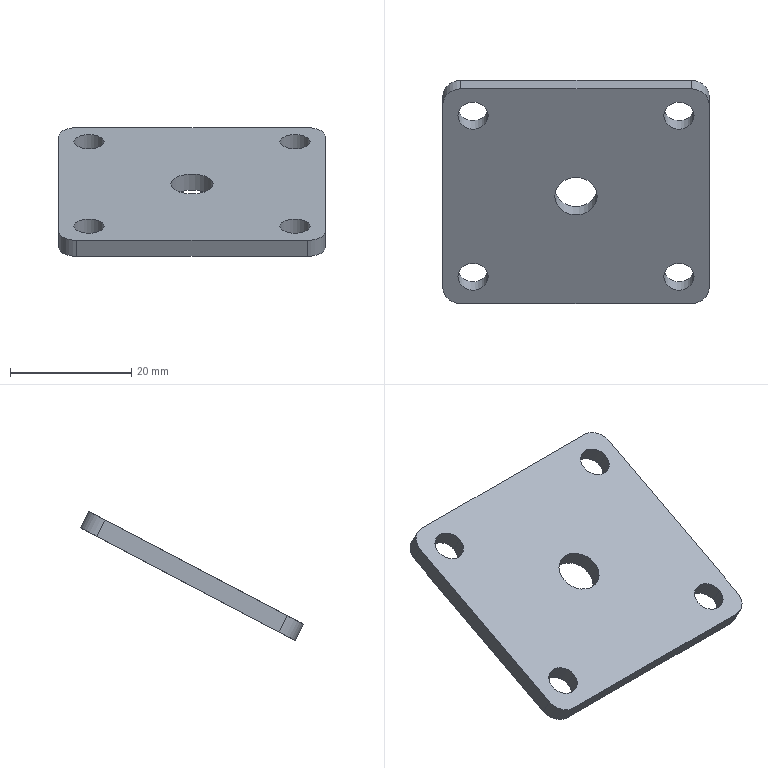Component | SolidWorks | SDACylinderPushPlate-1 | 1 solid | 20 faces | box 44 x 36.81 x 21.25 mm | volume 4906 mm3 | cylinder 14 | plane 6 | commonest cylinder face diameters 5 x8 6 x4 7 x2
STEP:
#1=COLOUR_RGB('',0.7922,0.8196,0.9333);
#2=FILL_AREA_STYLE_COLOUR('',#1);
#3=FILL_AREA_STYLE('',(#2));
#4=SURFACE_STYLE_FILL_AREA(#3);
#5=SURFACE_SIDE_STYLE('',(#4));
#6=SURFACE_STYLE_USAGE(.BOTH.,#5);
#7=PRESENTATION_STYLE_ASSIGNMENT((#6));
#8=CARTESIAN_POINT('',(-9.087,0.1913,6.018));
#9=VERTEX_POINT('',#8);
#10=CARTESIAN_POINT('',(-8.89,0.1913,6.018));
#11=VERTEX_POINT('',#10);
#12=CARTESIAN_POINT('',(-8.989,0.1913,6.018));
#13=DIRECTION('',(0.,-0.4648,0.8854));
#14=DIRECTION('',(1.,0.,0.));
#15=AXIS2_PLACEMENT_3D('',#12,#13,#14);
#16=CIRCLE('',#15,0.09843);
#17=EDGE_CURVE('',#9,#11,#16,.T.);
#18=ORIENTED_EDGE('',*,*,#17,.T.);
#19=CARTESIAN_POINT('',(-8.89,0.2462,5.913));
#20=VERTEX_POINT('',#19);
#21=CARTESIAN_POINT('',(-8.89,0.2462,5.913));
#22=DIRECTION('',(-0.,0.4648,-0.8854));
#23=VECTOR('',#22,39.37);
#24=LINE('',#21,#23);
#25=EDGE_CURVE('',#11,#20,#24,.T.);
#26=ORIENTED_EDGE('',*,*,#25,.T.);
#27=CARTESIAN_POINT('',(-9.087,0.2462,5.913));
#28=VERTEX_POINT('',#27);
#29=CARTESIAN_POINT('',(-8.989,0.2462,5.913));
#30=DIRECTION('',(-0.,0.4648,-0.8854));
#31=DIRECTION('',(-1.,-0.,0.));
#32=AXIS2_PLACEMENT_3D('',#29,#30,#31);
#33=CIRCLE('',#32,0.09843);
#34=EDGE_CURVE('',#20,#28,#33,.T.);
#35=ORIENTED_EDGE('',*,*,#34,.T.);
#36=CARTESIAN_POINT('',(-9.087,0.2462,5.913));
#37=DIRECTION('',(-0.,0.4648,-0.8854));
#38=VECTOR('',#37,39.37);
#39=LINE('',#36,#38);
#40=EDGE_CURVE('',#9,#28,#39,.T.);
#41=ORIENTED_EDGE('',*,*,#40,.F.);
#42=EDGE_LOOP('',(#18,#26,#35,#41));
#43=FACE_OUTER_BOUND('',#42,.T.);
#44=CARTESIAN_POINT('',(-8.989,0.2462,5.913));
#45=DIRECTION('',(-0.,0.4648,-0.8854));
#46=DIRECTION('',(-1.,-0.,0.));
#47=AXIS2_PLACEMENT_3D('',#44,#45,#46);
#48=CYLINDRICAL_SURFACE('',#47,0.09843);
#49=ADVANCED_FACE('',(#43),#48,.F.);
#50=CARTESIAN_POINT('',(-10.426,0.1913,6.018));
#51=VERTEX_POINT('',#50);
#52=CARTESIAN_POINT('',(-10.229,0.1913,6.018));
#53=VERTEX_POINT('',#52);
#54=CARTESIAN_POINT('',(-10.327,0.1913,6.018));
#55=DIRECTION('',(0.,-0.4648,0.8854));
#56=DIRECTION('',(1.,0.,0.));
#57=AXIS2_PLACEMENT_3D('',#54,#55,#56);
#58=CIRCLE('',#57,0.09843);
#59=EDGE_CURVE('',#51,#53,#58,.T.);
#60=ORIENTED_EDGE('',*,*,#59,.T.);
#61=CARTESIAN_POINT('',(-10.229,0.2462,5.913));
#62=VERTEX_POINT('',#61);
#63=CARTESIAN_POINT('',(-10.229,0.2462,5.913));
#64=DIRECTION('',(-0.,0.4648,-0.8854));
#65=VECTOR('',#64,39.37);
#66=LINE('',#63,#65);
#67=EDGE_CURVE('',#53,#62,#66,.T.);
#68=ORIENTED_EDGE('',*,*,#67,.T.);
#69=CARTESIAN_POINT('',(-10.426,0.2462,5.913));
#70=VERTEX_POINT('',#69);
#71=CARTESIAN_POINT('',(-10.327,0.2462,5.913));
#72=DIRECTION('',(-0.,0.4648,-0.8854));
#73=DIRECTION('',(-1.,-0.,0.));
#74=AXIS2_PLACEMENT_3D('',#71,#72,#73);
#75=CIRCLE('',#74,0.09843);
#76=EDGE_CURVE('',#62,#70,#75,.T.);
#77=ORIENTED_EDGE('',*,*,#76,.T.);
#78=CARTESIAN_POINT('',(-10.426,0.2462,5.913));
#79=DIRECTION('',(-0.,0.4648,-0.8854));
#80=VECTOR('',#79,39.37);
#81=LINE('',#78,#80);
#82=EDGE_CURVE('',#51,#70,#81,.T.);
#83=ORIENTED_EDGE('',*,*,#82,.F.);
#84=EDGE_LOOP('',(#60,#68,#77,#83));
#85=FACE_OUTER_BOUND('',#84,.T.);
#86=CARTESIAN_POINT('',(-10.327,0.2462,5.913));
#87=DIRECTION('',(-0.,0.4648,-0.8854));
#88=DIRECTION('',(-1.,-0.,0.));
#89=AXIS2_PLACEMENT_3D('',#86,#87,#88);
#90=CYLINDRICAL_SURFACE('',#89,0.09843);
#91=ADVANCED_FACE('',(#85),#90,.F.);
#92=CARTESIAN_POINT('',(-9.087,-0.8544,5.469));
#93=VERTEX_POINT('',#92);
#94=CARTESIAN_POINT('',(-8.89,-0.8544,5.469));
#95=VERTEX_POINT('',#94);
#96=CARTESIAN_POINT('',(-8.989,-0.8544,5.469));
#97=DIRECTION('',(0.,-0.4648,0.8854));
#98=DIRECTION('',(1.,0.,0.));
#99=AXIS2_PLACEMENT_3D('',#96,#97,#98);
#100=CIRCLE('',#99,0.09843);
#101=EDGE_CURVE('',#93,#95,#100,.T.);
#102=ORIENTED_EDGE('',*,*,#101,.T.);
#103=CARTESIAN_POINT('',(-8.89,-0.7995,5.364));
#104=VERTEX_POINT('',#103);
#105=CARTESIAN_POINT('',(-8.89,-0.7995,5.364));
#106=DIRECTION('',(-0.,0.4648,-0.8854));
#107=VECTOR('',#106,39.37);
#108=LINE('',#105,#107);
#109=EDGE_CURVE('',#95,#104,#108,.T.);
#110=ORIENTED_EDGE('',*,*,#109,.T.);
#111=CARTESIAN_POINT('',(-9.087,-0.7995,5.364));
#112=VERTEX_POINT('',#111);
#113=CARTESIAN_POINT('',(-8.989,-0.7995,5.364));
#114=DIRECTION('',(-0.,0.4648,-0.8854));
#115=DIRECTION('',(-1.,-0.,0.));
#116=AXIS2_PLACEMENT_3D('',#113,#114,#115);
#117=CIRCLE('',#116,0.09843);
#118=EDGE_CURVE('',#104,#112,#117,.T.);
#119=ORIENTED_EDGE('',*,*,#118,.T.);
#120=CARTESIAN_POINT('',(-9.087,-0.7995,5.364));
#121=DIRECTION('',(-0.,0.4648,-0.8854));
#122=VECTOR('',#121,39.37);
#123=LINE('',#120,#122);
#124=EDGE_CURVE('',#93,#112,#123,.T.);
#125=ORIENTED_EDGE('',*,*,#124,.F.);
#126=EDGE_LOOP('',(#102,#110,#119,#125));
#127=FACE_OUTER_BOUND('',#126,.T.);
#128=CARTESIAN_POINT('',(-8.989,-0.7995,5.364));
#129=DIRECTION('',(-0.,0.4648,-0.8854));
#130=DIRECTION('',(-1.,-0.,0.));
#131=AXIS2_PLACEMENT_3D('',#128,#129,#130);
#132=CYLINDRICAL_SURFACE('',#131,0.09843);
#133=ADVANCED_FACE('',(#127),#132,.F.);
#134=CARTESIAN_POINT('',(-10.426,-0.8544,5.469));
#135=VERTEX_POINT('',#134);
#136=CARTESIAN_POINT('',(-10.229,-0.8544,5.469));
#137=VERTEX_POINT('',#136);
#138=CARTESIAN_POINT('',(-10.327,-0.8544,5.469));
#139=DIRECTION('',(0.,-0.4648,0.8854));
#140=DIRECTION('',(1.,0.,0.));
#141=AXIS2_PLACEMENT_3D('',#138,#139,#140);
#142=CIRCLE('',#141,0.09843);
#143=EDGE_CURVE('',#135,#137,#142,.T.);
#144=ORIENTED_EDGE('',*,*,#143,.T.);
#145=CARTESIAN_POINT('',(-10.229,-0.7995,5.364));
#146=VERTEX_POINT('',#145);
#147=CARTESIAN_POINT('',(-10.229,-0.7995,5.364));
#148=DIRECTION('',(-0.,0.4648,-0.8854));
#149=VECTOR('',#148,39.37);
#150=LINE('',#147,#149);
#151=EDGE_CURVE('',#137,#146,#150,.T.);
#152=ORIENTED_EDGE('',*,*,#151,.T.);
#153=CARTESIAN_POINT('',(-10.426,-0.7995,5.364));
#154=VERTEX_POINT('',#153);
#155=CARTESIAN_POINT('',(-10.327,-0.7995,5.364));
#156=DIRECTION('',(-0.,0.4648,-0.8854));
#157=DIRECTION('',(-1.,-0.,0.));
#158=AXIS2_PLACEMENT_3D('',#155,#156,#157);
#159=CIRCLE('',#158,0.09843);
#160=EDGE_CURVE('',#146,#154,#159,.T.);
#161=ORIENTED_EDGE('',*,*,#160,.T.);
#162=CARTESIAN_POINT('',(-10.426,-0.7995,5.364));
#163=DIRECTION('',(-0.,0.4648,-0.8854));
#164=VECTOR('',#163,39.37);
#165=LINE('',#162,#164);
#166=EDGE_CURVE('',#135,#154,#165,.T.);
#167=ORIENTED_EDGE('',*,*,#166,.F.);
#168=EDGE_LOOP('',(#144,#152,#161,#167));
#169=FACE_OUTER_BOUND('',#168,.T.);
#170=CARTESIAN_POINT('',(-10.327,-0.7995,5.364));
#171=DIRECTION('',(-0.,0.4648,-0.8854));
#172=DIRECTION('',(-1.,-0.,0.));
#173=AXIS2_PLACEMENT_3D('',#170,#171,#172);
#174=CYLINDRICAL_SURFACE('',#173,0.09843);
#175=ADVANCED_FACE('',(#169),#174,.F.);
#176=CARTESIAN_POINT('',(-9.796,-0.3316,5.743));
#177=VERTEX_POINT('',#176);
#178=CARTESIAN_POINT('',(-9.52,-0.3316,5.743));
#179=VERTEX_POINT('',#178);
#180=CARTESIAN_POINT('',(-9.658,-0.3316,5.743));
#181=DIRECTION('',(0.,-0.4648,0.8854));
#182=DIRECTION('',(1.,0.,0.));
#183=AXIS2_PLACEMENT_3D('',#180,#181,#182);
#184=CIRCLE('',#183,0.1378);
#185=EDGE_CURVE('',#177,#179,#184,.T.);
#186=ORIENTED_EDGE('',*,*,#185,.T.);
#187=CARTESIAN_POINT('',(-9.52,-0.2767,5.638));
#188=VERTEX_POINT('',#187);
#189=CARTESIAN_POINT('',(-9.52,-0.2767,5.638));
#190=DIRECTION('',(-0.,0.4648,-0.8854));
#191=VECTOR('',#190,39.37);
#192=LINE('',#189,#191);
#193=EDGE_CURVE('',#179,#188,#192,.T.);
#194=ORIENTED_EDGE('',*,*,#193,.T.);
#195=CARTESIAN_POINT('',(-9.796,-0.2767,5.638));
#196=VERTEX_POINT('',#195);
#197=CARTESIAN_POINT('',(-9.658,-0.2767,5.638));
#198=DIRECTION('',(-0.,0.4648,-0.8854));
#199=DIRECTION('',(-1.,-0.,0.));
#200=AXIS2_PLACEMENT_3D('',#197,#198,#199);
#201=CIRCLE('',#200,0.1378);
#202=EDGE_CURVE('',#188,#196,#201,.T.);
#203=ORIENTED_EDGE('',*,*,#202,.T.);
#204=CARTESIAN_POINT('',(-9.796,-0.2767,5.638));
#205=DIRECTION('',(-0.,0.4648,-0.8854));
#206=VECTOR('',#205,39.37);
#207=LINE('',#204,#206);
#208=EDGE_CURVE('',#177,#196,#207,.T.);
#209=ORIENTED_EDGE('',*,*,#208,.F.);
#210=EDGE_LOOP('',(#186,#194,#203,#209));
#211=FACE_OUTER_BOUND('',#210,.T.);
#212=CARTESIAN_POINT('',(-9.658,-0.2767,5.638));
#213=DIRECTION('',(-0.,0.4648,-0.8854));
#214=DIRECTION('',(-1.,-0.,0.));
#215=AXIS2_PLACEMENT_3D('',#212,#213,#214);
#216=CYLINDRICAL_SURFACE('',#215,0.1378);
#217=ADVANCED_FACE('',(#211),#216,.F.);
#218=CARTESIAN_POINT('',(-10.524,-0.9242,5.432));
#219=VERTEX_POINT('',#218);
#220=CARTESIAN_POINT('',(-10.524,0.261,6.054));
#221=VERTEX_POINT('',#220);
#222=CARTESIAN_POINT('',(-10.524,-1.029,5.377));
#223=DIRECTION('',(-0.,0.8854,0.4648));
#224=VECTOR('',#223,39.37);
#225=LINE('',#222,#224);
#226=EDGE_CURVE('',#219,#221,#225,.T.);
#227=ORIENTED_EDGE('',*,*,#226,.T.);
#228=CARTESIAN_POINT('',(-10.524,0.3159,5.95));
#229=VERTEX_POINT('',#228);
#230=CARTESIAN_POINT('',(-10.524,0.261,6.054));
#231=DIRECTION('',(-0.,0.4648,-0.8854));
#232=VECTOR('',#231,39.37);
#233=LINE('',#230,#232);
#234=EDGE_CURVE('',#221,#229,#233,.T.);
#235=ORIENTED_EDGE('',*,*,#234,.T.);
#236=CARTESIAN_POINT('',(-10.524,-0.8693,5.327));
#237=VERTEX_POINT('',#236);
#238=CARTESIAN_POINT('',(-10.524,-0.9738,5.272));
#239=DIRECTION('',(-0.,0.8854,0.4648));
#240=VECTOR('',#239,39.37);
#241=LINE('',#238,#240);
#242=EDGE_CURVE('',#237,#229,#241,.T.);
#243=ORIENTED_EDGE('',*,*,#242,.F.);
#244=CARTESIAN_POINT('',(-10.524,-0.9242,5.432));
#245=DIRECTION('',(0.,-0.4648,0.8854));
#246=VECTOR('',#245,39.37);
#247=LINE('',#244,#246);
#248=EDGE_CURVE('',#237,#219,#247,.T.);
#249=ORIENTED_EDGE('',*,*,#248,.T.);
#250=EDGE_LOOP('',(#227,#235,#243,#249));
#251=FACE_OUTER_BOUND('',#250,.T.);
#252=CARTESIAN_POINT('',(-10.524,-1.029,5.377));
#253=DIRECTION('',(-1.,-0.,0.));
#254=DIRECTION('',(0.,-0.4648,0.8854));
#255=AXIS2_PLACEMENT_3D('',#252,#253,#254);
#256=PLANE('',#255);
#257=ADVANCED_FACE('',(#251),#256,.T.);
#258=CARTESIAN_POINT('',(-8.91,-1.029,5.377));
#259=VERTEX_POINT('',#258);
#260=CARTESIAN_POINT('',(-10.406,-1.029,5.377));
#261=VERTEX_POINT('',#260);
#262=CARTESIAN_POINT('',(-8.792,-1.029,5.377));
#263=DIRECTION('',(-1.,-0.,0.));
#264=VECTOR('',#263,39.37);
#265=LINE('',#262,#264);
#266=EDGE_CURVE('',#259,#261,#265,.T.);
#267=ORIENTED_EDGE('',*,*,#266,.T.);
#268=CARTESIAN_POINT('',(-10.406,-0.9738,5.272));
#269=VERTEX_POINT('',#268);
#270=CARTESIAN_POINT('',(-10.406,-1.029,5.377));
#271=DIRECTION('',(-0.,0.4648,-0.8854));
#272=VECTOR('',#271,39.37);
#273=LINE('',#270,#272);
#274=EDGE_CURVE('',#261,#269,#273,.T.);
#275=ORIENTED_EDGE('',*,*,#274,.T.);
#276=CARTESIAN_POINT('',(-8.91,-0.9738,5.272));
#277=VERTEX_POINT('',#276);
#278=CARTESIAN_POINT('',(-8.792,-0.9738,5.272));
#279=DIRECTION('',(-1.,-0.,0.));
#280=VECTOR('',#279,39.37);
#281=LINE('',#278,#280);
#282=EDGE_CURVE('',#277,#269,#281,.T.);
#283=ORIENTED_EDGE('',*,*,#282,.F.);
#284=CARTESIAN_POINT('',(-8.91,-1.029,5.377));
#285=DIRECTION('',(0.,-0.4648,0.8854));
#286=VECTOR('',#285,39.37);
#287=LINE('',#284,#286);
#288=EDGE_CURVE('',#277,#259,#287,.T.);
#289=ORIENTED_EDGE('',*,*,#288,.T.);
#290=EDGE_LOOP('',(#267,#275,#283,#289));
#291=FACE_OUTER_BOUND('',#290,.T.);
#292=CARTESIAN_POINT('',(-8.792,-1.029,5.377));
#293=DIRECTION('',(0.,-0.8854,-0.4648));
#294=DIRECTION('',(0.,-0.4648,0.8854));
#295=AXIS2_PLACEMENT_3D('',#292,#293,#294);
#296=PLANE('',#295);
#297=ADVANCED_FACE('',(#291),#296,.T.);
#298=CARTESIAN_POINT('',(-8.792,0.261,6.054));
#299=VERTEX_POINT('',#298);
#300=CARTESIAN_POINT('',(-8.792,-0.9242,5.432));
#301=VERTEX_POINT('',#300);
#302=CARTESIAN_POINT('',(-8.792,-1.029,5.377));
#303=DIRECTION('',(0.,-0.8854,-0.4648));
#304=VECTOR('',#303,39.37);
#305=LINE('',#302,#304);
#306=EDGE_CURVE('',#299,#301,#305,.T.);
#307=ORIENTED_EDGE('',*,*,#306,.T.);
#308=CARTESIAN_POINT('',(-8.792,-0.8693,5.327));
#309=VERTEX_POINT('',#308);
#310=CARTESIAN_POINT('',(-8.792,-0.9242,5.432));
#311=DIRECTION('',(-0.,0.4648,-0.8854));
#312=VECTOR('',#311,39.37);
#313=LINE('',#310,#312);
#314=EDGE_CURVE('',#301,#309,#313,.T.);
#315=ORIENTED_EDGE('',*,*,#314,.T.);
#316=CARTESIAN_POINT('',(-8.792,0.3159,5.95));
#317=VERTEX_POINT('',#316);
#318=CARTESIAN_POINT('',(-8.792,-0.9738,5.272));
#319=DIRECTION('',(0.,-0.8854,-0.4648));
#320=VECTOR('',#319,39.37);
#321=LINE('',#318,#320);
#322=EDGE_CURVE('',#317,#309,#321,.T.);
#323=ORIENTED_EDGE('',*,*,#322,.F.);
#324=CARTESIAN_POINT('',(-8.792,0.261,6.054));
#325=DIRECTION('',(0.,-0.4648,0.8854));
#326=VECTOR('',#325,39.37);
#327=LINE('',#324,#326);
#328=EDGE_CURVE('',#317,#299,#327,.T.);
#329=ORIENTED_EDGE('',*,*,#328,.T.);
#330=EDGE_LOOP('',(#307,#315,#323,#329));
#331=FACE_OUTER_BOUND('',#330,.T.);
#332=CARTESIAN_POINT('',(-8.792,-1.029,5.377));
#333=DIRECTION('',(1.,0.,-0.));
#334=DIRECTION('',(-0.,0.4648,-0.8854));
#335=AXIS2_PLACEMENT_3D('',#332,#333,#334);
#336=PLANE('',#335);
#337=ADVANCED_FACE('',(#331),#336,.T.);
#338=CARTESIAN_POINT('',(-10.406,0.4205,6.004));
#339=VERTEX_POINT('',#338);
#340=CARTESIAN_POINT('',(-8.91,0.4205,6.004));
#341=VERTEX_POINT('',#340);
#342=CARTESIAN_POINT('',(-8.792,0.4205,6.004));
#343=DIRECTION('',(1.,0.,-0.));
#344=VECTOR('',#343,39.37);
#345=LINE('',#342,#344);
#346=EDGE_CURVE('',#339,#341,#345,.T.);
#347=ORIENTED_EDGE('',*,*,#346,.F.);
#348=CARTESIAN_POINT('',(-10.406,0.3656,6.109));
#349=VERTEX_POINT('',#348);
#350=CARTESIAN_POINT('',(-10.406,0.3656,6.109));
#351=DIRECTION('',(0.,-0.4648,0.8854));
#352=VECTOR('',#351,39.37);
#353=LINE('',#350,#352);
#354=EDGE_CURVE('',#339,#349,#353,.T.);
#355=ORIENTED_EDGE('',*,*,#354,.T.);
#356=CARTESIAN_POINT('',(-8.91,0.3656,6.109));
#357=VERTEX_POINT('',#356);
#358=CARTESIAN_POINT('',(-8.792,0.3656,6.109));
#359=DIRECTION('',(1.,0.,-0.));
#360=VECTOR('',#359,39.37);
#361=LINE('',#358,#360);
#362=EDGE_CURVE('',#349,#357,#361,.T.);
#363=ORIENTED_EDGE('',*,*,#362,.T.);
#364=CARTESIAN_POINT('',(-8.91,0.3656,6.109));
#365=DIRECTION('',(-0.,0.4648,-0.8854));
#366=VECTOR('',#365,39.37);
#367=LINE('',#364,#366);
#368=EDGE_CURVE('',#357,#341,#367,.T.);
#369=ORIENTED_EDGE('',*,*,#368,.T.);
#370=EDGE_LOOP('',(#347,#355,#363,#369));
#371=FACE_OUTER_BOUND('',#370,.T.);
#372=CARTESIAN_POINT('',(-8.792,0.3656,6.109));
#373=DIRECTION('',(-0.,0.8854,0.4648));
#374=DIRECTION('',(-0.,0.4648,-0.8854));
#375=AXIS2_PLACEMENT_3D('',#372,#373,#374);
#376=PLANE('',#375);
#377=ADVANCED_FACE('',(#371),#376,.T.);
#378=ORIENTED_EDGE('',*,*,#17,.F.);
#379=CARTESIAN_POINT('',(-8.989,0.1913,6.018));
#380=DIRECTION('',(0.,-0.4648,0.8854));
#381=DIRECTION('',(1.,0.,0.));
#382=AXIS2_PLACEMENT_3D('',#379,#380,#381);
#383=CIRCLE('',#382,0.09843);
#384=EDGE_CURVE('',#11,#9,#383,.T.);
#385=ORIENTED_EDGE('',*,*,#384,.F.);
#386=EDGE_LOOP('',(#378,#385));
#387=FACE_BOUND('',#386,.T.);
#388=ORIENTED_EDGE('',*,*,#59,.F.);
#389=CARTESIAN_POINT('',(-10.327,0.1913,6.018));
#390=DIRECTION('',(0.,-0.4648,0.8854));
#391=DIRECTION('',(1.,0.,0.));
#392=AXIS2_PLACEMENT_3D('',#389,#390,#391);
#393=CIRCLE('',#392,0.09843);
#394=EDGE_CURVE('',#53,#51,#393,.T.);
#395=ORIENTED_EDGE('',*,*,#394,.F.);
#396=EDGE_LOOP('',(#388,#395));
#397=FACE_BOUND('',#396,.T.);
#398=ORIENTED_EDGE('',*,*,#101,.F.);
#399=CARTESIAN_POINT('',(-8.989,-0.8544,5.469));
#400=DIRECTION('',(0.,-0.4648,0.8854));
#401=DIRECTION('',(1.,0.,0.));
#402=AXIS2_PLACEMENT_3D('',#399,#400,#401);
#403=CIRCLE('',#402,0.09843);
#404=EDGE_CURVE('',#95,#93,#403,.T.);
#405=ORIENTED_EDGE('',*,*,#404,.F.);
#406=EDGE_LOOP('',(#398,#405));
#407=FACE_BOUND('',#406,.T.);
#408=ORIENTED_EDGE('',*,*,#143,.F.);
#409=CARTESIAN_POINT('',(-10.327,-0.8544,5.469));
#410=DIRECTION('',(0.,-0.4648,0.8854));
#411=DIRECTION('',(1.,0.,0.));
#412=AXIS2_PLACEMENT_3D('',#409,#410,#411);
#413=CIRCLE('',#412,0.09843);
#414=EDGE_CURVE('',#137,#135,#413,.T.);
#415=ORIENTED_EDGE('',*,*,#414,.F.);
#416=EDGE_LOOP('',(#408,#415));
#417=FACE_BOUND('',#416,.T.);
#418=ORIENTED_EDGE('',*,*,#185,.F.);
#419=CARTESIAN_POINT('',(-9.658,-0.3316,5.743));
#420=DIRECTION('',(0.,-0.4648,0.8854));
#421=DIRECTION('',(1.,0.,0.));
#422=AXIS2_PLACEMENT_3D('',#419,#420,#421);
#423=CIRCLE('',#422,0.1378);
#424=EDGE_CURVE('',#179,#177,#423,.T.);
#425=ORIENTED_EDGE('',*,*,#424,.F.);
#426=EDGE_LOOP('',(#418,#425));
#427=FACE_BOUND('',#426,.T.);
#428=ORIENTED_EDGE('',*,*,#362,.F.);
#429=CARTESIAN_POINT('',(-10.406,0.261,6.054));
#430=DIRECTION('',(0.,-0.4648,0.8854));
#431=DIRECTION('',(1.,0.,0.));
#432=AXIS2_PLACEMENT_3D('',#429,#430,#431);
#433=CIRCLE('',#432,0.1181);
#434=EDGE_CURVE('',#349,#221,#433,.T.);
#435=ORIENTED_EDGE('',*,*,#434,.T.);
#436=ORIENTED_EDGE('',*,*,#226,.F.);
#437=CARTESIAN_POINT('',(-10.406,-0.9242,5.432));
#438=DIRECTION('',(0.,-0.4648,0.8854));
#439=DIRECTION('',(1.,0.,0.));
#440=AXIS2_PLACEMENT_3D('',#437,#438,#439);
#441=CIRCLE('',#440,0.1181);
#442=EDGE_CURVE('',#219,#261,#441,.T.);
#443=ORIENTED_EDGE('',*,*,#442,.T.);
#444=ORIENTED_EDGE('',*,*,#266,.F.);
#445=CARTESIAN_POINT('',(-8.91,-0.9242,5.432));
#446=DIRECTION('',(0.,-0.4648,0.8854));
#447=DIRECTION('',(1.,0.,0.));
#448=AXIS2_PLACEMENT_3D('',#445,#446,#447);
#449=CIRCLE('',#448,0.1181);
#450=EDGE_CURVE('',#259,#301,#449,.T.);
#451=ORIENTED_EDGE('',*,*,#450,.T.);
#452=ORIENTED_EDGE('',*,*,#306,.F.);
#453=CARTESIAN_POINT('',(-8.91,0.261,6.054));
#454=DIRECTION('',(0.,-0.4648,0.8854));
#455=DIRECTION('',(1.,0.,0.));
#456=AXIS2_PLACEMENT_3D('',#453,#454,#455);
#457=CIRCLE('',#456,0.1181);
#458=EDGE_CURVE('',#299,#357,#457,.T.);
#459=ORIENTED_EDGE('',*,*,#458,.T.);
#460=EDGE_LOOP('',(#428,#435,#436,#443,#444,#451,#452,#459));
#461=FACE_OUTER_BOUND('',#460,.T.);
#462=CARTESIAN_POINT('',(-9.658,-0.3316,5.743));
#463=DIRECTION('',(0.,-0.4648,0.8854));
#464=DIRECTION('',(1.,0.,-0.));
#465=AXIS2_PLACEMENT_3D('',#462,#463,#464);
#466=PLANE('',#465);
#467=ADVANCED_FACE('',(#387,#397,#407,#417,#427,#461),#466,.T.);
#468=CARTESIAN_POINT('',(-8.989,0.2462,5.913));
#469=DIRECTION('',(-0.,0.4648,-0.8854));
#470=DIRECTION('',(-1.,-0.,0.));
#471=AXIS2_PLACEMENT_3D('',#468,#469,#470);
#472=CIRCLE('',#471,0.09843);
#473=EDGE_CURVE('',#28,#20,#472,.T.);
#474=ORIENTED_EDGE('',*,*,#473,.F.);
#475=ORIENTED_EDGE('',*,*,#34,.F.);
#476=EDGE_LOOP('',(#474,#475));
#477=FACE_BOUND('',#476,.T.);
#478=CARTESIAN_POINT('',(-10.327,0.2462,5.913));
#479=DIRECTION('',(-0.,0.4648,-0.8854));
#480=DIRECTION('',(-1.,-0.,0.));
#481=AXIS2_PLACEMENT_3D('',#478,#479,#480);
#482=CIRCLE('',#481,0.09843);
#483=EDGE_CURVE('',#70,#62,#482,.T.);
#484=ORIENTED_EDGE('',*,*,#483,.F.);
#485=ORIENTED_EDGE('',*,*,#76,.F.);
#486=EDGE_LOOP('',(#484,#485));
#487=FACE_BOUND('',#486,.T.);
#488=CARTESIAN_POINT('',(-8.989,-0.7995,5.364));
#489=DIRECTION('',(-0.,0.4648,-0.8854));
#490=DIRECTION('',(-1.,-0.,0.));
#491=AXIS2_PLACEMENT_3D('',#488,#489,#490);
#492=CIRCLE('',#491,0.09843);
#493=EDGE_CURVE('',#112,#104,#492,.T.);
#494=ORIENTED_EDGE('',*,*,#493,.F.);
#495=ORIENTED_EDGE('',*,*,#118,.F.);
#496=EDGE_LOOP('',(#494,#495));
#497=FACE_BOUND('',#496,.T.);
#498=CARTESIAN_POINT('',(-10.327,-0.7995,5.364));
#499=DIRECTION('',(-0.,0.4648,-0.8854));
#500=DIRECTION('',(-1.,-0.,0.));
#501=AXIS2_PLACEMENT_3D('',#498,#499,#500);
#502=CIRCLE('',#501,0.09843);
#503=EDGE_CURVE('',#154,#146,#502,.T.);
#504=ORIENTED_EDGE('',*,*,#503,.F.);
#505=ORIENTED_EDGE('',*,*,#160,.F.);
#506=EDGE_LOOP('',(#504,#505));
#507=FACE_BOUND('',#506,.T.);
#508=CARTESIAN_POINT('',(-9.658,-0.2767,5.638));
#509=DIRECTION('',(-0.,0.4648,-0.8854));
#510=DIRECTION('',(-1.,-0.,0.));
#511=AXIS2_PLACEMENT_3D('',#508,#509,#510);
#512=CIRCLE('',#511,0.1378);
#513=EDGE_CURVE('',#196,#188,#512,.T.);
#514=ORIENTED_EDGE('',*,*,#513,.F.);
#515=ORIENTED_EDGE('',*,*,#202,.F.);
#516=EDGE_LOOP('',(#514,#515));
#517=FACE_BOUND('',#516,.T.);
#518=ORIENTED_EDGE('',*,*,#242,.T.);
#519=CARTESIAN_POINT('',(-10.406,0.3159,5.95));
#520=DIRECTION('',(-0.,0.4648,-0.8854));
#521=DIRECTION('',(1.,0.,0.));
#522=AXIS2_PLACEMENT_3D('',#519,#520,#521);
#523=CIRCLE('',#522,0.1181);
#524=EDGE_CURVE('',#229,#339,#523,.T.);
#525=ORIENTED_EDGE('',*,*,#524,.T.);
#526=ORIENTED_EDGE('',*,*,#346,.T.);
#527=CARTESIAN_POINT('',(-8.91,0.3159,5.95));
#528=DIRECTION('',(-0.,0.4648,-0.8854));
#529=DIRECTION('',(1.,0.,0.));
#530=AXIS2_PLACEMENT_3D('',#527,#528,#529);
#531=CIRCLE('',#530,0.1181);
#532=EDGE_CURVE('',#341,#317,#531,.T.);
#533=ORIENTED_EDGE('',*,*,#532,.T.);
#534=ORIENTED_EDGE('',*,*,#322,.T.);
#535=CARTESIAN_POINT('',(-8.91,-0.8693,5.327));
#536=DIRECTION('',(-0.,0.4648,-0.8854));
#537=DIRECTION('',(1.,0.,0.));
#538=AXIS2_PLACEMENT_3D('',#535,#536,#537);
#539=CIRCLE('',#538,0.1181);
#540=EDGE_CURVE('',#309,#277,#539,.T.);
#541=ORIENTED_EDGE('',*,*,#540,.T.);
#542=ORIENTED_EDGE('',*,*,#282,.T.);
#543=CARTESIAN_POINT('',(-10.406,-0.8693,5.327));
#544=DIRECTION('',(-0.,0.4648,-0.8854));
#545=DIRECTION('',(1.,0.,0.));
#546=AXIS2_PLACEMENT_3D('',#543,#544,#545);
#547=CIRCLE('',#546,0.1181);
#548=EDGE_CURVE('',#269,#237,#547,.T.);
#549=ORIENTED_EDGE('',*,*,#548,.T.);
#550=EDGE_LOOP('',(#518,#525,#526,#533,#534,#541,#542,#549));
#551=FACE_OUTER_BOUND('',#550,.T.);
#552=CARTESIAN_POINT('',(-9.658,-0.2767,5.638));
#553=DIRECTION('',(0.,-0.4648,0.8854));
#554=DIRECTION('',(1.,0.,-0.));
#555=AXIS2_PLACEMENT_3D('',#552,#553,#554);
#556=PLANE('',#555);
#557=ADVANCED_FACE('',(#477,#487,#497,#507,#517,#551),#556,.F.);
#558=ORIENTED_EDGE('',*,*,#193,.F.);
#559=ORIENTED_EDGE('',*,*,#424,.T.);
#560=ORIENTED_EDGE('',*,*,#208,.T.);
#561=ORIENTED_EDGE('',*,*,#513,.T.);
#562=EDGE_LOOP('',(#558,#559,#560,#561));
#563=FACE_OUTER_BOUND('',#562,.T.);
#564=CARTESIAN_POINT('',(-9.658,-0.2767,5.638));
#565=DIRECTION('',(-0.,0.4648,-0.8854));
#566=DIRECTION('',(-1.,-0.,0.));
#567=AXIS2_PLACEMENT_3D('',#564,#565,#566);
#568=CYLINDRICAL_SURFACE('',#567,0.1378);
#569=ADVANCED_FACE('',(#563),#568,.F.);
#570=ORIENTED_EDGE('',*,*,#151,.F.);
#571=ORIENTED_EDGE('',*,*,#414,.T.);
#572=ORIENTED_EDGE('',*,*,#166,.T.);
#573=ORIENTED_EDGE('',*,*,#503,.T.);
#574=EDGE_LOOP('',(#570,#571,#572,#573));
#575=FACE_OUTER_BOUND('',#574,.T.);
#576=CARTESIAN_POINT('',(-10.327,-0.7995,5.364));
#577=DIRECTION('',(-0.,0.4648,-0.8854));
#578=DIRECTION('',(-1.,-0.,0.));
#579=AXIS2_PLACEMENT_3D('',#576,#577,#578);
#580=CYLINDRICAL_SURFACE('',#579,0.09843);
#581=ADVANCED_FACE('',(#575),#580,.F.);
#582=ORIENTED_EDGE('',*,*,#109,.F.);
#583=ORIENTED_EDGE('',*,*,#404,.T.);
#584=ORIENTED_EDGE('',*,*,#124,.T.);
#585=ORIENTED_EDGE('',*,*,#493,.T.);
#586=EDGE_LOOP('',(#582,#583,#584,#585));
#587=FACE_OUTER_BOUND('',#586,.T.);
#588=CARTESIAN_POINT('',(-8.989,-0.7995,5.364));
#589=DIRECTION('',(-0.,0.4648,-0.8854));
#590=DIRECTION('',(-1.,-0.,0.));
#591=AXIS2_PLACEMENT_3D('',#588,#589,#590);
#592=CYLINDRICAL_SURFACE('',#591,0.09843);
#593=ADVANCED_FACE('',(#587),#592,.F.);
#594=ORIENTED_EDGE('',*,*,#67,.F.);
#595=ORIENTED_EDGE('',*,*,#394,.T.);
#596=ORIENTED_EDGE('',*,*,#82,.T.);
#597=ORIENTED_EDGE('',*,*,#483,.T.);
#598=EDGE_LOOP('',(#594,#595,#596,#597));
#599=FACE_OUTER_BOUND('',#598,.T.);
#600=CARTESIAN_POINT('',(-10.327,0.2462,5.913));
#601=DIRECTION('',(-0.,0.4648,-0.8854));
#602=DIRECTION('',(-1.,-0.,0.));
#603=AXIS2_PLACEMENT_3D('',#600,#601,#602);
#604=CYLINDRICAL_SURFACE('',#603,0.09843);
#605=ADVANCED_FACE('',(#599),#604,.F.);
#606=ORIENTED_EDGE('',*,*,#25,.F.);
#607=ORIENTED_EDGE('',*,*,#384,.T.);
#608=ORIENTED_EDGE('',*,*,#40,.T.);
#609=ORIENTED_EDGE('',*,*,#473,.T.);
#610=EDGE_LOOP('',(#606,#607,#608,#609));
#611=FACE_OUTER_BOUND('',#610,.T.);
#612=CARTESIAN_POINT('',(-8.989,0.2462,5.913));
#613=DIRECTION('',(-0.,0.4648,-0.8854));
#614=DIRECTION('',(-1.,-0.,0.));
#615=AXIS2_PLACEMENT_3D('',#612,#613,#614);
#616=CYLINDRICAL_SURFACE('',#615,0.09843);
#617=ADVANCED_FACE('',(#611),#616,.F.);
#618=ORIENTED_EDGE('',*,*,#434,.F.);
#619=ORIENTED_EDGE('',*,*,#354,.F.);
#620=ORIENTED_EDGE('',*,*,#524,.F.);
#621=ORIENTED_EDGE('',*,*,#234,.F.);
#622=EDGE_LOOP('',(#618,#619,#620,#621));
#623=FACE_OUTER_BOUND('',#622,.T.);
#624=CARTESIAN_POINT('',(-10.406,0.261,6.054));
#625=DIRECTION('',(-0.,0.4648,-0.8854));
#626=DIRECTION('',(-1.,-0.,0.));
#627=AXIS2_PLACEMENT_3D('',#624,#625,#626);
#628=CYLINDRICAL_SURFACE('',#627,0.1181);
#629=ADVANCED_FACE('',(#623),#628,.T.);
#630=ORIENTED_EDGE('',*,*,#442,.F.);
#631=ORIENTED_EDGE('',*,*,#248,.F.);
#632=ORIENTED_EDGE('',*,*,#548,.F.);
#633=ORIENTED_EDGE('',*,*,#274,.F.);
#634=EDGE_LOOP('',(#630,#631,#632,#633));
#635=FACE_OUTER_BOUND('',#634,.T.);
#636=CARTESIAN_POINT('',(-10.406,-0.9242,5.432));
#637=DIRECTION('',(-0.,0.4648,-0.8854));
#638=DIRECTION('',(-1.,-0.,0.));
#639=AXIS2_PLACEMENT_3D('',#636,#637,#638);
#640=CYLINDRICAL_SURFACE('',#639,0.1181);
#641=ADVANCED_FACE('',(#635),#640,.T.);
#642=ORIENTED_EDGE('',*,*,#450,.F.);
#643=ORIENTED_EDGE('',*,*,#288,.F.);
#644=ORIENTED_EDGE('',*,*,#540,.F.);
#645=ORIENTED_EDGE('',*,*,#314,.F.);
#646=EDGE_LOOP('',(#642,#643,#644,#645));
#647=FACE_OUTER_BOUND('',#646,.T.);
#648=CARTESIAN_POINT('',(-8.91,-0.9242,5.432));
#649=DIRECTION('',(-0.,0.4648,-0.8854));
#650=DIRECTION('',(-1.,-0.,0.));
#651=AXIS2_PLACEMENT_3D('',#648,#649,#650);
#652=CYLINDRICAL_SURFACE('',#651,0.1181);
#653=ADVANCED_FACE('',(#647),#652,.T.);
#654=ORIENTED_EDGE('',*,*,#458,.F.);
#655=ORIENTED_EDGE('',*,*,#328,.F.);
#656=ORIENTED_EDGE('',*,*,#532,.F.);
#657=ORIENTED_EDGE('',*,*,#368,.F.);
#658=EDGE_LOOP('',(#654,#655,#656,#657));
#659=FACE_OUTER_BOUND('',#658,.T.);
#660=CARTESIAN_POINT('',(-8.91,0.261,6.054));
#661=DIRECTION('',(-0.,0.4648,-0.8854));
#662=DIRECTION('',(-1.,-0.,0.));
#663=AXIS2_PLACEMENT_3D('',#660,#661,#662);
#664=CYLINDRICAL_SURFACE('',#663,0.1181);
#665=ADVANCED_FACE('',(#659),#664,.T.);
#666=CLOSED_SHELL('',(#49,#91,#133,#175,#217,#257,#297,#337,#377,#467,#557,#569,#581,#593,#605,#617,#629,#641,#653,#665));
#667=MANIFOLD_SOLID_BREP('',#666);
#668=STYLED_ITEM('',(#7),#667);
#669=(LENGTH_UNIT()NAMED_UNIT(*)SI_UNIT($,.METRE.));
#670=LENGTH_MEASURE_WITH_UNIT(LENGTH_MEASURE(0.0254),#669);
#671=DIMENSIONAL_EXPONENTS(1.,0.,0.,0.,0.,0.,0.);
#672=(CONVERSION_BASED_UNIT('',#670)LENGTH_UNIT()NAMED_UNIT(#671));
#673=UNCERTAINTY_MEASURE_WITH_UNIT(LENGTH_MEASURE(0.00001),#672,'','');
#674=(NAMED_UNIT(*)PLANE_ANGLE_UNIT()SI_UNIT($,.RADIAN.));
#675=(NAMED_UNIT(*)SI_UNIT($,.STERADIAN.)SOLID_ANGLE_UNIT());
#676=(GEOMETRIC_REPRESENTATION_CONTEXT(3)GLOBAL_UNCERTAINTY_ASSIGNED_CONTEXT((#673))GLOBAL_UNIT_ASSIGNED_CONTEXT((#672,#674,#675))REPRESENTATION_CONTEXT('',''));
#677=MECHANICAL_DESIGN_GEOMETRIC_PRESENTATION_REPRESENTATION('',(#668),#676);
#678=CARTESIAN_POINT('',(0.,0.,0.));
#679=DIRECTION('',(0.,0.,1.));
#680=DIRECTION('',(1.,0.,0.));
#681=AXIS2_PLACEMENT_3D('',#678,#679,#680);
#682=(LENGTH_UNIT()NAMED_UNIT(*)SI_UNIT($,.METRE.));
#683=LENGTH_MEASURE_WITH_UNIT(LENGTH_MEASURE(0.0254),#682);
#684=DIMENSIONAL_EXPONENTS(1.,0.,0.,0.,0.,0.,0.);
#685=(CONVERSION_BASED_UNIT('',#683)LENGTH_UNIT()NAMED_UNIT(#684));
#686=UNCERTAINTY_MEASURE_WITH_UNIT(LENGTH_MEASURE(0.00001),#685,'','');
#687=(NAMED_UNIT(*)PLANE_ANGLE_UNIT()SI_UNIT($,.RADIAN.));
#688=(NAMED_UNIT(*)SI_UNIT($,.STERADIAN.)SOLID_ANGLE_UNIT());
#689=(GEOMETRIC_REPRESENTATION_CONTEXT(3)GLOBAL_UNCERTAINTY_ASSIGNED_CONTEXT((#686))GLOBAL_UNIT_ASSIGNED_CONTEXT((#685,#687,#688))REPRESENTATION_CONTEXT('',''));
#690=ADVANCED_BREP_SHAPE_REPRESENTATION('',(#667,#681),#689);
#691=PRESENTATION_LAYER_ASSIGNMENT('','',(#668));